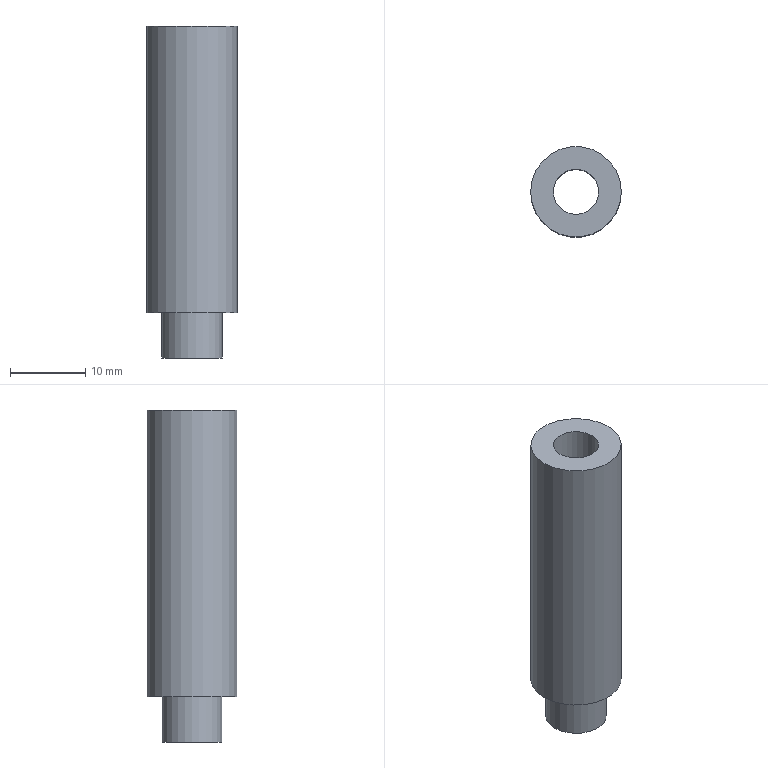Component | NX | BREATHER_PIPE | 1 solid | 6 faces | volume 3355 mm3 | plane 3 | cylinder 3 | commonest cylinder face diameters 8 x1 12 x1 6 x1